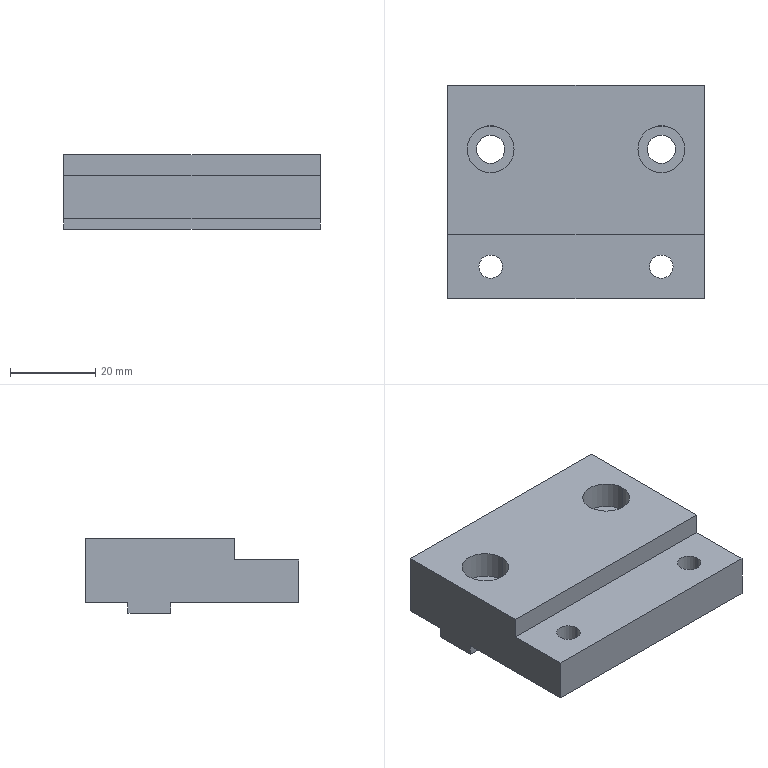Component | SolidWorks | Q1-A12-S21-Q4E.SLDASQ-4_Q1-A12-S21-Q4E-01A-1 | 1 solid | 32 faces | box 60 x 50 x 17.5 mm | volume 38957 mm3 | cylinder 16 | plane 16 | commonest cylinder face diameters 10 x4 5.5 x4 11 x4 6.6 x4 | material Q235-Steel
build123d program:
from build123d import *

# Parameters (mm, degrees)
SKETCH1_W                                       = 60
SKETCH1_H                                       = 50
BOSS_EXTRUDE1_DEPTH                             = 17.5
SKETCH2_W                                       = 5
SKETCH2_H                                       = 15
CUT_EXTRUDE1_DEPTH                              = 68.315
M6_HEX_SOCKET_HEAD_CAP_SCREW_CBORE2_D           = 6.6
M6_HEX_SOCKET_HEAD_CAP_SCREW_CBORE2_CBORE_D     = 11
M6_HEX_SOCKET_HEAD_CAP_SCREW_CBORE2_CBORE_DEPTH = 6.4
SKETCH7_W                                       = 2.5
SKETCH7_H                                       = 10
SKETCH7_H_2                                     = 30
CUT_EXTRUDE2_DEPTH                              = 68.315
M5_HEX_SOCKET_HEAD_CAP_SCREW_CBORE1_D           = 5.5
M5_HEX_SOCKET_HEAD_CAP_SCREW_CBORE1_CBORE_D     = 10
M5_HEX_SOCKET_HEAD_CAP_SCREW_CBORE1_CBORE_DEPTH = 5.4


with BuildPart() as part:
    # Sketch1 → Boss-Extrude1 (new body)
    with BuildSketch(Plane.XY):
        Rectangle(SKETCH1_W, SKETCH1_H)
    extrude(amount=BOSS_EXTRUDE1_DEPTH)

    # Sketch2 → Cut-Extrude1 (cut, through all)
    with BuildSketch(Plane(origin=(30, 0, 0), x_dir=(0, 0, -1), z_dir=(1, 0, 0))):
        with Locations((-15, -17.5)):
            Rectangle(SKETCH2_W, SKETCH2_H)
    extrude(amount=-CUT_EXTRUDE1_DEPTH, mode=Mode.SUBTRACT)

    # M6 Hex Socket Head Cap Screw CBORE2 (through all)
    with Locations(Plane.XY.offset(17.5)):
        with Locations((20, 10), (-20, 10)):
            CounterBoreHole(M6_HEX_SOCKET_HEAD_CAP_SCREW_CBORE2_D / 2, M6_HEX_SOCKET_HEAD_CAP_SCREW_CBORE2_CBORE_D / 2, M6_HEX_SOCKET_HEAD_CAP_SCREW_CBORE2_CBORE_DEPTH)

    # Sketch7 → Cut-Extrude2 (cut, through all)
    with BuildSketch(Plane(origin=(30, 0, 0), x_dir=(0, 0, -1), z_dir=(1, 0, 0))):
        with Locations((-1.25, 20)):
            Rectangle(SKETCH7_W, SKETCH7_H)
        with Locations((-1.25, -10)):
            Rectangle(SKETCH7_W, SKETCH7_H_2)
    extrude(amount=-CUT_EXTRUDE2_DEPTH, mode=Mode.SUBTRACT)

    # M5 Hex Socket Head Cap Screw CBORE1 (through all)
    with Locations(Plane(origin=(0, 0, 2.5), x_dir=(-1, 0, 0), z_dir=(0, 0, -1))):
        with Locations((-20, -17.5), (20, -17.5)):
            CounterBoreHole(M5_HEX_SOCKET_HEAD_CAP_SCREW_CBORE1_D / 2, M5_HEX_SOCKET_HEAD_CAP_SCREW_CBORE1_CBORE_D / 2, M5_HEX_SOCKET_HEAD_CAP_SCREW_CBORE1_CBORE_DEPTH)


solid = part.part

# Placed as in the assembly
solid = solid.moved(Location((1798.5, -30, 147.5), (0, 0, 0)))
STEP:
#1=COLOUR_RGB('',0.7922,0.8196,0.9333);
#2=FILL_AREA_STYLE_COLOUR('',#1);
#3=FILL_AREA_STYLE('',(#2));
#4=SURFACE_STYLE_FILL_AREA(#3);
#5=SURFACE_SIDE_STYLE('',(#4));
#6=SURFACE_STYLE_USAGE(.BOTH.,#5);
#7=PRESENTATION_STYLE_ASSIGNMENT((#6));
#8=CARTESIAN_POINT('',(71.791,-1.87,6.118));
#9=VERTEX_POINT('',#8);
#10=CARTESIAN_POINT('',(71.398,-1.87,6.118));
#11=VERTEX_POINT('',#10);
#12=CARTESIAN_POINT('',(71.594,-1.87,6.118));
#13=DIRECTION('',(0.,0.,-1.));
#14=DIRECTION('',(-1.,0.,0.));
#15=AXIS2_PLACEMENT_3D('',#12,#13,#14);
#16=CIRCLE('',#15,0.1969);
#17=EDGE_CURVE('',#9,#11,#16,.T.);
#18=ORIENTED_EDGE('',*,*,#17,.F.);
#19=CARTESIAN_POINT('',(71.791,-1.87,5.906));
#20=VERTEX_POINT('',#19);
#21=CARTESIAN_POINT('',(71.791,-1.87,5.906));
#22=DIRECTION('',(0.,0.,-1.));
#23=VECTOR('',#22,39.37);
#24=LINE('',#21,#23);
#25=EDGE_CURVE('',#9,#20,#24,.T.);
#26=ORIENTED_EDGE('',*,*,#25,.T.);
#27=CARTESIAN_POINT('',(71.398,-1.87,5.906));
#28=VERTEX_POINT('',#27);
#29=CARTESIAN_POINT('',(71.594,-1.87,5.906));
#30=DIRECTION('',(0.,0.,-1.));
#31=DIRECTION('',(-1.,0.,0.));
#32=AXIS2_PLACEMENT_3D('',#29,#30,#31);
#33=CIRCLE('',#32,0.1969);
#34=EDGE_CURVE('',#20,#28,#33,.T.);
#35=ORIENTED_EDGE('',*,*,#34,.T.);
#36=CARTESIAN_POINT('',(71.398,-1.87,5.906));
#37=DIRECTION('',(0.,0.,-1.));
#38=VECTOR('',#37,39.37);
#39=LINE('',#36,#38);
#40=EDGE_CURVE('',#11,#28,#39,.T.);
#41=ORIENTED_EDGE('',*,*,#40,.F.);
#42=EDGE_LOOP('',(#18,#26,#35,#41));
#43=FACE_OUTER_BOUND('',#42,.T.);
#44=CARTESIAN_POINT('',(71.594,-1.87,5.906));
#45=DIRECTION('',(0.,0.,-1.));
#46=DIRECTION('',(-1.,0.,0.));
#47=AXIS2_PLACEMENT_3D('',#44,#45,#46);
#48=CYLINDRICAL_SURFACE('',#47,0.1969);
#49=ADVANCED_FACE('',(#43),#48,.F.);
#50=CARTESIAN_POINT('',(71.703,-1.87,6.299));
#51=VERTEX_POINT('',#50);
#52=CARTESIAN_POINT('',(71.486,-1.87,6.299));
#53=VERTEX_POINT('',#52);
#54=CARTESIAN_POINT('',(71.594,-1.87,6.299));
#55=DIRECTION('',(0.,0.,-1.));
#56=DIRECTION('',(-1.,0.,0.));
#57=AXIS2_PLACEMENT_3D('',#54,#55,#56);
#58=CIRCLE('',#57,0.1083);
#59=EDGE_CURVE('',#51,#53,#58,.T.);
#60=ORIENTED_EDGE('',*,*,#59,.F.);
#61=CARTESIAN_POINT('',(71.703,-1.87,6.118));
#62=VERTEX_POINT('',#61);
#63=CARTESIAN_POINT('',(71.703,-1.87,5.906));
#64=DIRECTION('',(0.,0.,-1.));
#65=VECTOR('',#64,39.37);
#66=LINE('',#63,#65);
#67=EDGE_CURVE('',#51,#62,#66,.T.);
#68=ORIENTED_EDGE('',*,*,#67,.T.);
#69=CARTESIAN_POINT('',(71.486,-1.87,6.118));
#70=VERTEX_POINT('',#69);
#71=CARTESIAN_POINT('',(71.594,-1.87,6.118));
#72=DIRECTION('',(0.,0.,-1.));
#73=DIRECTION('',(-1.,0.,0.));
#74=AXIS2_PLACEMENT_3D('',#71,#72,#73);
#75=CIRCLE('',#74,0.1083);
#76=EDGE_CURVE('',#62,#70,#75,.T.);
#77=ORIENTED_EDGE('',*,*,#76,.T.);
#78=CARTESIAN_POINT('',(71.486,-1.87,5.906));
#79=DIRECTION('',(0.,0.,-1.));
#80=VECTOR('',#79,39.37);
#81=LINE('',#78,#80);
#82=EDGE_CURVE('',#53,#70,#81,.T.);
#83=ORIENTED_EDGE('',*,*,#82,.F.);
#84=EDGE_LOOP('',(#60,#68,#77,#83));
#85=FACE_OUTER_BOUND('',#84,.T.);
#86=CARTESIAN_POINT('',(71.594,-1.87,5.906));
#87=DIRECTION('',(0.,0.,-1.));
#88=DIRECTION('',(-1.,0.,0.));
#89=AXIS2_PLACEMENT_3D('',#86,#87,#88);
#90=CYLINDRICAL_SURFACE('',#89,0.1083);
#91=ADVANCED_FACE('',(#85),#90,.F.);
#92=CARTESIAN_POINT('',(70.217,-1.87,6.118));
#93=VERTEX_POINT('',#92);
#94=CARTESIAN_POINT('',(69.823,-1.87,6.118));
#95=VERTEX_POINT('',#94);
#96=CARTESIAN_POINT('',(70.02,-1.87,6.118));
#97=DIRECTION('',(0.,0.,-1.));
#98=DIRECTION('',(-1.,0.,0.));
#99=AXIS2_PLACEMENT_3D('',#96,#97,#98);
#100=CIRCLE('',#99,0.1969);
#101=EDGE_CURVE('',#93,#95,#100,.T.);
#102=ORIENTED_EDGE('',*,*,#101,.F.);
#103=CARTESIAN_POINT('',(70.217,-1.87,5.906));
#104=VERTEX_POINT('',#103);
#105=CARTESIAN_POINT('',(70.217,-1.87,5.906));
#106=DIRECTION('',(0.,0.,-1.));
#107=VECTOR('',#106,39.37);
#108=LINE('',#105,#107);
#109=EDGE_CURVE('',#93,#104,#108,.T.);
#110=ORIENTED_EDGE('',*,*,#109,.T.);
#111=CARTESIAN_POINT('',(69.823,-1.87,5.906));
#112=VERTEX_POINT('',#111);
#113=CARTESIAN_POINT('',(70.02,-1.87,5.906));
#114=DIRECTION('',(0.,0.,-1.));
#115=DIRECTION('',(-1.,0.,0.));
#116=AXIS2_PLACEMENT_3D('',#113,#114,#115);
#117=CIRCLE('',#116,0.1969);
#118=EDGE_CURVE('',#104,#112,#117,.T.);
#119=ORIENTED_EDGE('',*,*,#118,.T.);
#120=CARTESIAN_POINT('',(69.823,-1.87,5.906));
#121=DIRECTION('',(0.,0.,-1.));
#122=VECTOR('',#121,39.37);
#123=LINE('',#120,#122);
#124=EDGE_CURVE('',#95,#112,#123,.T.);
#125=ORIENTED_EDGE('',*,*,#124,.F.);
#126=EDGE_LOOP('',(#102,#110,#119,#125));
#127=FACE_OUTER_BOUND('',#126,.T.);
#128=CARTESIAN_POINT('',(70.02,-1.87,5.906));
#129=DIRECTION('',(0.,0.,-1.));
#130=DIRECTION('',(-1.,0.,0.));
#131=AXIS2_PLACEMENT_3D('',#128,#129,#130);
#132=CYLINDRICAL_SURFACE('',#131,0.1969);
#133=ADVANCED_FACE('',(#127),#132,.F.);
#134=CARTESIAN_POINT('',(70.128,-1.87,6.299));
#135=VERTEX_POINT('',#134);
#136=CARTESIAN_POINT('',(69.911,-1.87,6.299));
#137=VERTEX_POINT('',#136);
#138=CARTESIAN_POINT('',(70.02,-1.87,6.299));
#139=DIRECTION('',(0.,0.,-1.));
#140=DIRECTION('',(-1.,0.,0.));
#141=AXIS2_PLACEMENT_3D('',#138,#139,#140);
#142=CIRCLE('',#141,0.1083);
#143=EDGE_CURVE('',#135,#137,#142,.T.);
#144=ORIENTED_EDGE('',*,*,#143,.F.);
#145=CARTESIAN_POINT('',(70.128,-1.87,6.118));
#146=VERTEX_POINT('',#145);
#147=CARTESIAN_POINT('',(70.128,-1.87,5.906));
#148=DIRECTION('',(0.,0.,-1.));
#149=VECTOR('',#148,39.37);
#150=LINE('',#147,#149);
#151=EDGE_CURVE('',#135,#146,#150,.T.);
#152=ORIENTED_EDGE('',*,*,#151,.T.);
#153=CARTESIAN_POINT('',(69.911,-1.87,6.118));
#154=VERTEX_POINT('',#153);
#155=CARTESIAN_POINT('',(70.02,-1.87,6.118));
#156=DIRECTION('',(0.,0.,-1.));
#157=DIRECTION('',(-1.,0.,0.));
#158=AXIS2_PLACEMENT_3D('',#155,#156,#157);
#159=CIRCLE('',#158,0.1083);
#160=EDGE_CURVE('',#146,#154,#159,.T.);
#161=ORIENTED_EDGE('',*,*,#160,.T.);
#162=CARTESIAN_POINT('',(69.911,-1.87,5.906));
#163=DIRECTION('',(0.,0.,-1.));
#164=VECTOR('',#163,39.37);
#165=LINE('',#162,#164);
#166=EDGE_CURVE('',#137,#154,#165,.T.);
#167=ORIENTED_EDGE('',*,*,#166,.F.);
#168=EDGE_LOOP('',(#144,#152,#161,#167));
#169=FACE_OUTER_BOUND('',#168,.T.);
#170=CARTESIAN_POINT('',(70.02,-1.87,5.906));
#171=DIRECTION('',(0.,0.,-1.));
#172=DIRECTION('',(-1.,0.,0.));
#173=AXIS2_PLACEMENT_3D('',#170,#171,#172);
#174=CYLINDRICAL_SURFACE('',#173,0.1083);
#175=ADVANCED_FACE('',(#169),#174,.F.);
#176=CARTESIAN_POINT('',(71.378,-0.7874,6.244));
#177=VERTEX_POINT('',#176);
#178=CARTESIAN_POINT('',(71.811,-0.7874,6.244));
#179=VERTEX_POINT('',#178);
#180=CARTESIAN_POINT('',(71.594,-0.7874,6.244));
#181=DIRECTION('',(0.,0.,1.));
#182=DIRECTION('',(1.,0.,0.));
#183=AXIS2_PLACEMENT_3D('',#180,#181,#182);
#184=CIRCLE('',#183,0.2165);
#185=EDGE_CURVE('',#177,#179,#184,.T.);
#186=ORIENTED_EDGE('',*,*,#185,.F.);
#187=CARTESIAN_POINT('',(71.378,-0.7874,6.496));
#188=VERTEX_POINT('',#187);
#189=CARTESIAN_POINT('',(71.378,-0.7874,6.496));
#190=DIRECTION('',(0.,0.,1.));
#191=VECTOR('',#190,39.37);
#192=LINE('',#189,#191);
#193=EDGE_CURVE('',#177,#188,#192,.T.);
#194=ORIENTED_EDGE('',*,*,#193,.T.);
#195=CARTESIAN_POINT('',(71.811,-0.7874,6.496));
#196=VERTEX_POINT('',#195);
#197=CARTESIAN_POINT('',(71.594,-0.7874,6.496));
#198=DIRECTION('',(0.,0.,1.));
#199=DIRECTION('',(1.,0.,0.));
#200=AXIS2_PLACEMENT_3D('',#197,#198,#199);
#201=CIRCLE('',#200,0.2165);
#202=EDGE_CURVE('',#188,#196,#201,.T.);
#203=ORIENTED_EDGE('',*,*,#202,.T.);
#204=CARTESIAN_POINT('',(71.811,-0.7874,6.496));
#205=DIRECTION('',(0.,0.,1.));
#206=VECTOR('',#205,39.37);
#207=LINE('',#204,#206);
#208=EDGE_CURVE('',#179,#196,#207,.T.);
#209=ORIENTED_EDGE('',*,*,#208,.F.);
#210=EDGE_LOOP('',(#186,#194,#203,#209));
#211=FACE_OUTER_BOUND('',#210,.T.);
#212=CARTESIAN_POINT('',(71.594,-0.7874,6.496));
#213=DIRECTION('',(0.,0.,1.));
#214=DIRECTION('',(1.,0.,0.));
#215=AXIS2_PLACEMENT_3D('',#212,#213,#214);
#216=CYLINDRICAL_SURFACE('',#215,0.2165);
#217=ADVANCED_FACE('',(#211),#216,.F.);
#218=CARTESIAN_POINT('',(71.465,-0.7874,5.807));
#219=VERTEX_POINT('',#218);
#220=CARTESIAN_POINT('',(71.724,-0.7874,5.807));
#221=VERTEX_POINT('',#220);
#222=CARTESIAN_POINT('',(71.594,-0.7874,5.807));
#223=DIRECTION('',(0.,0.,1.));
#224=DIRECTION('',(1.,0.,0.));
#225=AXIS2_PLACEMENT_3D('',#222,#223,#224);
#226=CIRCLE('',#225,0.1299);
#227=EDGE_CURVE('',#219,#221,#226,.T.);
#228=ORIENTED_EDGE('',*,*,#227,.F.);
#229=CARTESIAN_POINT('',(71.465,-0.7874,6.244));
#230=VERTEX_POINT('',#229);
#231=CARTESIAN_POINT('',(71.465,-0.7874,6.496));
#232=DIRECTION('',(0.,0.,1.));
#233=VECTOR('',#232,39.37);
#234=LINE('',#231,#233);
#235=EDGE_CURVE('',#219,#230,#234,.T.);
#236=ORIENTED_EDGE('',*,*,#235,.T.);
#237=CARTESIAN_POINT('',(71.724,-0.7874,6.244));
#238=VERTEX_POINT('',#237);
#239=CARTESIAN_POINT('',(71.594,-0.7874,6.244));
#240=DIRECTION('',(0.,0.,1.));
#241=DIRECTION('',(1.,0.,0.));
#242=AXIS2_PLACEMENT_3D('',#239,#240,#241);
#243=CIRCLE('',#242,0.1299);
#244=EDGE_CURVE('',#230,#238,#243,.T.);
#245=ORIENTED_EDGE('',*,*,#244,.T.);
#246=CARTESIAN_POINT('',(71.724,-0.7874,6.496));
#247=DIRECTION('',(0.,0.,1.));
#248=VECTOR('',#247,39.37);
#249=LINE('',#246,#248);
#250=EDGE_CURVE('',#221,#238,#249,.T.);
#251=ORIENTED_EDGE('',*,*,#250,.F.);
#252=EDGE_LOOP('',(#228,#236,#245,#251));
#253=FACE_OUTER_BOUND('',#252,.T.);
#254=CARTESIAN_POINT('',(71.594,-0.7874,6.496));
#255=DIRECTION('',(0.,0.,1.));
#256=DIRECTION('',(1.,0.,0.));
#257=AXIS2_PLACEMENT_3D('',#254,#255,#256);
#258=CYLINDRICAL_SURFACE('',#257,0.1299);
#259=ADVANCED_FACE('',(#253),#258,.F.);
#260=CARTESIAN_POINT('',(69.803,-0.7874,6.244));
#261=VERTEX_POINT('',#260);
#262=CARTESIAN_POINT('',(70.236,-0.7874,6.244));
#263=VERTEX_POINT('',#262);
#264=CARTESIAN_POINT('',(70.02,-0.7874,6.244));
#265=DIRECTION('',(0.,0.,1.));
#266=DIRECTION('',(1.,0.,0.));
#267=AXIS2_PLACEMENT_3D('',#264,#265,#266);
#268=CIRCLE('',#267,0.2165);
#269=EDGE_CURVE('',#261,#263,#268,.T.);
#270=ORIENTED_EDGE('',*,*,#269,.F.);
#271=CARTESIAN_POINT('',(69.803,-0.7874,6.496));
#272=VERTEX_POINT('',#271);
#273=CARTESIAN_POINT('',(69.803,-0.7874,6.496));
#274=DIRECTION('',(0.,0.,1.));
#275=VECTOR('',#274,39.37);
#276=LINE('',#273,#275);
#277=EDGE_CURVE('',#261,#272,#276,.T.);
#278=ORIENTED_EDGE('',*,*,#277,.T.);
#279=CARTESIAN_POINT('',(70.236,-0.7874,6.496));
#280=VERTEX_POINT('',#279);
#281=CARTESIAN_POINT('',(70.02,-0.7874,6.496));
#282=DIRECTION('',(0.,0.,1.));
#283=DIRECTION('',(1.,0.,0.));
#284=AXIS2_PLACEMENT_3D('',#281,#282,#283);
#285=CIRCLE('',#284,0.2165);
#286=EDGE_CURVE('',#272,#280,#285,.T.);
#287=ORIENTED_EDGE('',*,*,#286,.T.);
#288=CARTESIAN_POINT('',(70.236,-0.7874,6.496));
#289=DIRECTION('',(0.,0.,1.));
#290=VECTOR('',#289,39.37);
#291=LINE('',#288,#290);
#292=EDGE_CURVE('',#263,#280,#291,.T.);
#293=ORIENTED_EDGE('',*,*,#292,.F.);
#294=EDGE_LOOP('',(#270,#278,#287,#293));
#295=FACE_OUTER_BOUND('',#294,.T.);
#296=CARTESIAN_POINT('',(70.02,-0.7874,6.496));
#297=DIRECTION('',(0.,0.,1.));
#298=DIRECTION('',(1.,0.,0.));
#299=AXIS2_PLACEMENT_3D('',#296,#297,#298);
#300=CYLINDRICAL_SURFACE('',#299,0.2165);
#301=ADVANCED_FACE('',(#295),#300,.F.);
#302=CARTESIAN_POINT('',(69.89,-0.7874,5.807));
#303=VERTEX_POINT('',#302);
#304=CARTESIAN_POINT('',(70.15,-0.7874,5.807));
#305=VERTEX_POINT('',#304);
#306=CARTESIAN_POINT('',(70.02,-0.7874,5.807));
#307=DIRECTION('',(0.,0.,1.));
#308=DIRECTION('',(1.,0.,0.));
#309=AXIS2_PLACEMENT_3D('',#306,#307,#308);
#310=CIRCLE('',#309,0.1299);
#311=EDGE_CURVE('',#303,#305,#310,.T.);
#312=ORIENTED_EDGE('',*,*,#311,.F.);
#313=CARTESIAN_POINT('',(69.89,-0.7874,6.244));
#314=VERTEX_POINT('',#313);
#315=CARTESIAN_POINT('',(69.89,-0.7874,6.496));
#316=DIRECTION('',(0.,0.,1.));
#317=VECTOR('',#316,39.37);
#318=LINE('',#315,#317);
#319=EDGE_CURVE('',#303,#314,#318,.T.);
#320=ORIENTED_EDGE('',*,*,#319,.T.);
#321=CARTESIAN_POINT('',(70.15,-0.7874,6.244));
#322=VERTEX_POINT('',#321);
#323=CARTESIAN_POINT('',(70.02,-0.7874,6.244));
#324=DIRECTION('',(0.,0.,1.));
#325=DIRECTION('',(1.,0.,0.));
#326=AXIS2_PLACEMENT_3D('',#323,#324,#325);
#327=CIRCLE('',#326,0.1299);
#328=EDGE_CURVE('',#314,#322,#327,.T.);
#329=ORIENTED_EDGE('',*,*,#328,.T.);
#330=CARTESIAN_POINT('',(70.15,-0.7874,6.496));
#331=DIRECTION('',(0.,0.,1.));
#332=VECTOR('',#331,39.37);
#333=LINE('',#330,#332);
#334=EDGE_CURVE('',#305,#322,#333,.T.);
#335=ORIENTED_EDGE('',*,*,#334,.F.);
#336=EDGE_LOOP('',(#312,#320,#329,#335));
#337=FACE_OUTER_BOUND('',#336,.T.);
#338=CARTESIAN_POINT('',(70.02,-0.7874,6.496));
#339=DIRECTION('',(0.,0.,1.));
#340=DIRECTION('',(1.,0.,0.));
#341=AXIS2_PLACEMENT_3D('',#338,#339,#340);
#342=CYLINDRICAL_SURFACE('',#341,0.1299);
#343=ADVANCED_FACE('',(#337),#342,.F.);
#344=CARTESIAN_POINT('',(71.988,-2.165,6.299));
#345=VERTEX_POINT('',#344);
#346=CARTESIAN_POINT('',(71.988,-2.165,5.906));
#347=VERTEX_POINT('',#346);
#348=CARTESIAN_POINT('',(71.988,-2.165,6.496));
#349=DIRECTION('',(0.,0.,-1.));
#350=VECTOR('',#349,39.37);
#351=LINE('',#348,#350);
#352=EDGE_CURVE('',#345,#347,#351,.T.);
#353=ORIENTED_EDGE('',*,*,#352,.T.);
#354=CARTESIAN_POINT('',(71.988,-0.9843,5.906));
#355=VERTEX_POINT('',#354);
#356=CARTESIAN_POINT('',(71.988,-2.165,5.906));
#357=DIRECTION('',(0.,-1.,0.));
#358=VECTOR('',#357,39.37);
#359=LINE('',#356,#358);
#360=EDGE_CURVE('',#355,#347,#359,.T.);
#361=ORIENTED_EDGE('',*,*,#360,.F.);
#362=CARTESIAN_POINT('',(71.988,-0.9843,5.807));
#363=VERTEX_POINT('',#362);
#364=CARTESIAN_POINT('',(71.988,-0.9843,5.807));
#365=DIRECTION('',(0.,0.,1.));
#366=VECTOR('',#365,39.37);
#367=LINE('',#364,#366);
#368=EDGE_CURVE('',#363,#355,#367,.T.);
#369=ORIENTED_EDGE('',*,*,#368,.F.);
#370=CARTESIAN_POINT('',(71.988,-0.5906,5.807));
#371=VERTEX_POINT('',#370);
#372=CARTESIAN_POINT('',(71.988,-2.165,5.807));
#373=DIRECTION('',(0.,1.,0.));
#374=VECTOR('',#373,39.37);
#375=LINE('',#372,#374);
#376=EDGE_CURVE('',#363,#371,#375,.T.);
#377=ORIENTED_EDGE('',*,*,#376,.T.);
#378=CARTESIAN_POINT('',(71.988,-0.5906,5.906));
#379=VERTEX_POINT('',#378);
#380=CARTESIAN_POINT('',(71.988,-0.5906,5.807));
#381=DIRECTION('',(0.,0.,-1.));
#382=VECTOR('',#381,39.37);
#383=LINE('',#380,#382);
#384=EDGE_CURVE('',#379,#371,#383,.T.);
#385=ORIENTED_EDGE('',*,*,#384,.F.);
#386=CARTESIAN_POINT('',(71.988,-0.1969,5.906));
#387=VERTEX_POINT('',#386);
#388=CARTESIAN_POINT('',(71.988,-0.1969,5.906));
#389=DIRECTION('',(0.,-1.,0.));
#390=VECTOR('',#389,39.37);
#391=LINE('',#388,#390);
#392=EDGE_CURVE('',#387,#379,#391,.T.);
#393=ORIENTED_EDGE('',*,*,#392,.F.);
#394=CARTESIAN_POINT('',(71.988,-0.1969,6.496));
#395=VERTEX_POINT('',#394);
#396=CARTESIAN_POINT('',(71.988,-0.1969,6.496));
#397=DIRECTION('',(0.,0.,-1.));
#398=VECTOR('',#397,39.37);
#399=LINE('',#396,#398);
#400=EDGE_CURVE('',#395,#387,#399,.T.);
#401=ORIENTED_EDGE('',*,*,#400,.F.);
#402=CARTESIAN_POINT('',(71.988,-1.575,6.496));
#403=VERTEX_POINT('',#402);
#404=CARTESIAN_POINT('',(71.988,-2.165,6.496));
#405=DIRECTION('',(0.,1.,0.));
#406=VECTOR('',#405,39.37);
#407=LINE('',#404,#406);
#408=EDGE_CURVE('',#403,#395,#407,.T.);
#409=ORIENTED_EDGE('',*,*,#408,.F.);
#410=CARTESIAN_POINT('',(71.988,-1.575,6.299));
#411=VERTEX_POINT('',#410);
#412=CARTESIAN_POINT('',(71.988,-1.575,6.496));
#413=DIRECTION('',(0.,0.,1.));
#414=VECTOR('',#413,39.37);
#415=LINE('',#412,#414);
#416=EDGE_CURVE('',#411,#403,#415,.T.);
#417=ORIENTED_EDGE('',*,*,#416,.F.);
#418=CARTESIAN_POINT('',(71.988,-2.165,6.299));
#419=DIRECTION('',(0.,1.,0.));
#420=VECTOR('',#419,39.37);
#421=LINE('',#418,#420);
#422=EDGE_CURVE('',#345,#411,#421,.T.);
#423=ORIENTED_EDGE('',*,*,#422,.F.);
#424=EDGE_LOOP('',(#353,#361,#369,#377,#385,#393,#401,#409,#417,#423));
#425=FACE_OUTER_BOUND('',#424,.T.);
#426=CARTESIAN_POINT('',(71.988,-2.165,6.496));
#427=DIRECTION('',(-1.,0.,0.));
#428=DIRECTION('',(0.,0.,1.));
#429=AXIS2_PLACEMENT_3D('',#426,#427,#428);
#430=PLANE('',#429);
#431=ADVANCED_FACE('',(#425),#430,.F.);
#432=ORIENTED_EDGE('',*,*,#400,.T.);
#433=CARTESIAN_POINT('',(69.626,-0.1969,5.906));
#434=VERTEX_POINT('',#433);
#435=CARTESIAN_POINT('',(69.626,-0.1969,5.906));
#436=DIRECTION('',(1.,0.,0.));
#437=VECTOR('',#436,39.37);
#438=LINE('',#435,#437);
#439=EDGE_CURVE('',#434,#387,#438,.T.);
#440=ORIENTED_EDGE('',*,*,#439,.F.);
#441=CARTESIAN_POINT('',(69.626,-0.1969,6.496));
#442=VERTEX_POINT('',#441);
#443=CARTESIAN_POINT('',(69.626,-0.1969,6.496));
#444=DIRECTION('',(0.,0.,-1.));
#445=VECTOR('',#444,39.37);
#446=LINE('',#443,#445);
#447=EDGE_CURVE('',#442,#434,#446,.T.);
#448=ORIENTED_EDGE('',*,*,#447,.F.);
#449=CARTESIAN_POINT('',(69.626,-0.1969,6.496));
#450=DIRECTION('',(-1.,0.,0.));
#451=VECTOR('',#450,39.37);
#452=LINE('',#449,#451);
#453=EDGE_CURVE('',#395,#442,#452,.T.);
#454=ORIENTED_EDGE('',*,*,#453,.F.);
#455=EDGE_LOOP('',(#432,#440,#448,#454));
#456=FACE_OUTER_BOUND('',#455,.T.);
#457=CARTESIAN_POINT('',(69.626,-0.1969,6.496));
#458=DIRECTION('',(0.,-1.,0.));
#459=DIRECTION('',(0.,0.,-1.));
#460=AXIS2_PLACEMENT_3D('',#457,#458,#459);
#461=PLANE('',#460);
#462=ADVANCED_FACE('',(#456),#461,.F.);
#463=CARTESIAN_POINT('',(69.626,-0.9843,5.807));
#464=VERTEX_POINT('',#463);
#465=CARTESIAN_POINT('',(69.626,-0.9843,5.906));
#466=VERTEX_POINT('',#465);
#467=CARTESIAN_POINT('',(69.626,-0.9843,5.807));
#468=DIRECTION('',(0.,0.,1.));
#469=VECTOR('',#468,39.37);
#470=LINE('',#467,#469);
#471=EDGE_CURVE('',#464,#466,#470,.T.);
#472=ORIENTED_EDGE('',*,*,#471,.T.);
#473=CARTESIAN_POINT('',(69.626,-2.165,5.906));
#474=VERTEX_POINT('',#473);
#475=CARTESIAN_POINT('',(69.626,-2.165,5.906));
#476=DIRECTION('',(0.,-1.,0.));
#477=VECTOR('',#476,39.37);
#478=LINE('',#475,#477);
#479=EDGE_CURVE('',#466,#474,#478,.T.);
#480=ORIENTED_EDGE('',*,*,#479,.T.);
#481=CARTESIAN_POINT('',(69.626,-2.165,6.299));
#482=VERTEX_POINT('',#481);
#483=CARTESIAN_POINT('',(69.626,-2.165,6.496));
#484=DIRECTION('',(0.,0.,-1.));
#485=VECTOR('',#484,39.37);
#486=LINE('',#483,#485);
#487=EDGE_CURVE('',#482,#474,#486,.T.);
#488=ORIENTED_EDGE('',*,*,#487,.F.);
#489=CARTESIAN_POINT('',(69.626,-1.575,6.299));
#490=VERTEX_POINT('',#489);
#491=CARTESIAN_POINT('',(69.626,-2.165,6.299));
#492=DIRECTION('',(0.,1.,0.));
#493=VECTOR('',#492,39.37);
#494=LINE('',#491,#493);
#495=EDGE_CURVE('',#482,#490,#494,.T.);
#496=ORIENTED_EDGE('',*,*,#495,.T.);
#497=CARTESIAN_POINT('',(69.626,-1.575,6.496));
#498=VERTEX_POINT('',#497);
#499=CARTESIAN_POINT('',(69.626,-1.575,6.496));
#500=DIRECTION('',(0.,0.,1.));
#501=VECTOR('',#500,39.37);
#502=LINE('',#499,#501);
#503=EDGE_CURVE('',#490,#498,#502,.T.);
#504=ORIENTED_EDGE('',*,*,#503,.T.);
#505=CARTESIAN_POINT('',(69.626,-2.165,6.496));
#506=DIRECTION('',(0.,-1.,0.));
#507=VECTOR('',#506,39.37);
#508=LINE('',#505,#507);
#509=EDGE_CURVE('',#442,#498,#508,.T.);
#510=ORIENTED_EDGE('',*,*,#509,.F.);
#511=ORIENTED_EDGE('',*,*,#447,.T.);
#512=CARTESIAN_POINT('',(69.626,-0.5906,5.906));
#513=VERTEX_POINT('',#512);
#514=CARTESIAN_POINT('',(69.626,-0.1969,5.906));
#515=DIRECTION('',(0.,-1.,0.));
#516=VECTOR('',#515,39.37);
#517=LINE('',#514,#516);
#518=EDGE_CURVE('',#434,#513,#517,.T.);
#519=ORIENTED_EDGE('',*,*,#518,.T.);
#520=CARTESIAN_POINT('',(69.626,-0.5906,5.807));
#521=VERTEX_POINT('',#520);
#522=CARTESIAN_POINT('',(69.626,-0.5906,5.807));
#523=DIRECTION('',(0.,0.,-1.));
#524=VECTOR('',#523,39.37);
#525=LINE('',#522,#524);
#526=EDGE_CURVE('',#513,#521,#525,.T.);
#527=ORIENTED_EDGE('',*,*,#526,.T.);
#528=CARTESIAN_POINT('',(69.626,-2.165,5.807));
#529=DIRECTION('',(0.,-1.,0.));
#530=VECTOR('',#529,39.37);
#531=LINE('',#528,#530);
#532=EDGE_CURVE('',#521,#464,#531,.T.);
#533=ORIENTED_EDGE('',*,*,#532,.T.);
#534=EDGE_LOOP('',(#472,#480,#488,#496,#504,#510,#511,#519,#527,#533));
#535=FACE_OUTER_BOUND('',#534,.T.);
#536=CARTESIAN_POINT('',(69.626,-2.165,6.496));
#537=DIRECTION('',(1.,0.,0.));
#538=DIRECTION('',(0.,0.,-1.));
#539=AXIS2_PLACEMENT_3D('',#536,#537,#538);
#540=PLANE('',#539);
#541=ADVANCED_FACE('',(#535),#540,.F.);
#542=ORIENTED_EDGE('',*,*,#487,.T.);
#543=CARTESIAN_POINT('',(69.626,-2.165,5.906));
#544=DIRECTION('',(1.,0.,0.));
#545=VECTOR('',#544,39.37);
#546=LINE('',#543,#545);
#547=EDGE_CURVE('',#474,#347,#546,.T.);
#548=ORIENTED_EDGE('',*,*,#547,.T.);
#549=ORIENTED_EDGE('',*,*,#352,.F.);
#550=CARTESIAN_POINT('',(69.626,-2.165,6.299));
#551=DIRECTION('',(1.,0.,0.));
#552=VECTOR('',#551,39.37);
#553=LINE('',#550,#552);
#554=EDGE_CURVE('',#482,#345,#553,.T.);
#555=ORIENTED_EDGE('',*,*,#554,.F.);
#556=EDGE_LOOP('',(#542,#548,#549,#555));
#557=FACE_OUTER_BOUND('',#556,.T.);
#558=CARTESIAN_POINT('',(69.626,-2.165,6.496));
#559=DIRECTION('',(0.,1.,0.));
#560=DIRECTION('',(0.,0.,1.));
#561=AXIS2_PLACEMENT_3D('',#558,#559,#560);
#562=PLANE('',#561);
#563=ADVANCED_FACE('',(#557),#562,.F.);
#564=CARTESIAN_POINT('',(71.594,-0.7874,6.496));
#565=DIRECTION('',(0.,0.,1.));
#566=DIRECTION('',(1.,0.,0.));
#567=AXIS2_PLACEMENT_3D('',#564,#565,#566);
#568=CIRCLE('',#567,0.2165);
#569=EDGE_CURVE('',#196,#188,#568,.T.);
#570=ORIENTED_EDGE('',*,*,#569,.F.);
#571=ORIENTED_EDGE('',*,*,#202,.F.);
#572=EDGE_LOOP('',(#570,#571));
#573=FACE_BOUND('',#572,.T.);
#574=CARTESIAN_POINT('',(70.02,-0.7874,6.496));
#575=DIRECTION('',(0.,0.,1.));
#576=DIRECTION('',(1.,0.,0.));
#577=AXIS2_PLACEMENT_3D('',#574,#575,#576);
#578=CIRCLE('',#577,0.2165);
#579=EDGE_CURVE('',#280,#272,#578,.T.);
#580=ORIENTED_EDGE('',*,*,#579,.F.);
#581=ORIENTED_EDGE('',*,*,#286,.F.);
#582=EDGE_LOOP('',(#580,#581));
#583=FACE_BOUND('',#582,.T.);
#584=ORIENTED_EDGE('',*,*,#509,.T.);
#585=CARTESIAN_POINT('',(69.626,-1.575,6.496));
#586=DIRECTION('',(1.,0.,0.));
#587=VECTOR('',#586,39.37);
#588=LINE('',#585,#587);
#589=EDGE_CURVE('',#498,#403,#588,.T.);
#590=ORIENTED_EDGE('',*,*,#589,.T.);
#591=ORIENTED_EDGE('',*,*,#408,.T.);
#592=ORIENTED_EDGE('',*,*,#453,.T.);
#593=EDGE_LOOP('',(#584,#590,#591,#592));
#594=FACE_OUTER_BOUND('',#593,.T.);
#595=CARTESIAN_POINT('',(70.807,-1.181,6.496));
#596=DIRECTION('',(0.,0.,-1.));
#597=DIRECTION('',(-1.,0.,0.));
#598=AXIS2_PLACEMENT_3D('',#595,#596,#597);
#599=PLANE('',#598);
#600=ADVANCED_FACE('',(#573,#583,#594),#599,.F.);
#601=CARTESIAN_POINT('',(69.626,-0.9843,5.807));
#602=DIRECTION('',(1.,0.,0.));
#603=VECTOR('',#602,39.37);
#604=LINE('',#601,#603);
#605=EDGE_CURVE('',#464,#363,#604,.T.);
#606=ORIENTED_EDGE('',*,*,#605,.F.);
#607=ORIENTED_EDGE('',*,*,#532,.F.);
#608=CARTESIAN_POINT('',(69.626,-0.5906,5.807));
#609=DIRECTION('',(1.,0.,0.));
#610=VECTOR('',#609,39.37);
#611=LINE('',#608,#610);
#612=EDGE_CURVE('',#521,#371,#611,.T.);
#613=ORIENTED_EDGE('',*,*,#612,.T.);
#614=ORIENTED_EDGE('',*,*,#376,.F.);
#615=EDGE_LOOP('',(#606,#607,#613,#614));
#616=FACE_OUTER_BOUND('',#615,.T.);
#617=CARTESIAN_POINT('',(71.594,-0.7874,5.807));
#618=DIRECTION('',(0.,0.,1.));
#619=DIRECTION('',(1.,0.,0.));
#620=AXIS2_PLACEMENT_3D('',#617,#618,#619);
#621=CIRCLE('',#620,0.1299);
#622=EDGE_CURVE('',#221,#219,#621,.T.);
#623=ORIENTED_EDGE('',*,*,#622,.T.);
#624=ORIENTED_EDGE('',*,*,#227,.T.);
#625=EDGE_LOOP('',(#623,#624));
#626=FACE_BOUND('',#625,.T.);
#627=CARTESIAN_POINT('',(70.02,-0.7874,5.807));
#628=DIRECTION('',(0.,0.,1.));
#629=DIRECTION('',(1.,0.,0.));
#630=AXIS2_PLACEMENT_3D('',#627,#628,#629);
#631=CIRCLE('',#630,0.1299);
#632=EDGE_CURVE('',#305,#303,#631,.T.);
#633=ORIENTED_EDGE('',*,*,#632,.T.);
#634=ORIENTED_EDGE('',*,*,#311,.T.);
#635=EDGE_LOOP('',(#633,#634));
#636=FACE_BOUND('',#635,.T.);
#637=CARTESIAN_POINT('',(70.807,-1.181,5.807));
#638=DIRECTION('',(0.,0.,-1.));
#639=DIRECTION('',(-1.,0.,0.));
#640=AXIS2_PLACEMENT_3D('',#637,#638,#639);
#641=PLANE('',#640);
#642=ADVANCED_FACE('',(#616,#626,#636),#641,.T.);
#643=ORIENTED_EDGE('',*,*,#416,.T.);
#644=ORIENTED_EDGE('',*,*,#589,.F.);
#645=ORIENTED_EDGE('',*,*,#503,.F.);
#646=CARTESIAN_POINT('',(69.626,-1.575,6.299));
#647=DIRECTION('',(1.,0.,0.));
#648=VECTOR('',#647,39.37);
#649=LINE('',#646,#648);
#650=EDGE_CURVE('',#490,#411,#649,.T.);
#651=ORIENTED_EDGE('',*,*,#650,.T.);
#652=EDGE_LOOP('',(#643,#644,#645,#651));
#653=FACE_OUTER_BOUND('',#652,.T.);
#654=CARTESIAN_POINT('',(69.626,-1.575,6.496));
#655=DIRECTION('',(0.,1.,0.));
#656=DIRECTION('',(0.,0.,1.));
#657=AXIS2_PLACEMENT_3D('',#654,#655,#656);
#658=PLANE('',#657);
#659=ADVANCED_FACE('',(#653),#658,.F.);
#660=CARTESIAN_POINT('',(71.594,-1.87,6.299));
#661=DIRECTION('',(0.,0.,-1.));
#662=DIRECTION('',(-1.,0.,0.));
#663=AXIS2_PLACEMENT_3D('',#660,#661,#662);
#664=CIRCLE('',#663,0.1083);
#665=EDGE_CURVE('',#53,#51,#664,.T.);
#666=ORIENTED_EDGE('',*,*,#665,.T.);
#667=ORIENTED_EDGE('',*,*,#59,.T.);
#668=EDGE_LOOP('',(#666,#667));
#669=FACE_BOUND('',#668,.T.);
#670=CARTESIAN_POINT('',(70.02,-1.87,6.299));
#671=DIRECTION('',(0.,0.,-1.));
#672=DIRECTION('',(-1.,0.,0.));
#673=AXIS2_PLACEMENT_3D('',#670,#671,#672);
#674=CIRCLE('',#673,0.1083);
#675=EDGE_CURVE('',#137,#135,#674,.T.);
#676=ORIENTED_EDGE('',*,*,#675,.T.);
#677=ORIENTED_EDGE('',*,*,#143,.T.);
#678=EDGE_LOOP('',(#676,#677));
#679=FACE_BOUND('',#678,.T.);
#680=ORIENTED_EDGE('',*,*,#422,.T.);
#681=ORIENTED_EDGE('',*,*,#650,.F.);
#682=ORIENTED_EDGE('',*,*,#495,.F.);
#683=ORIENTED_EDGE('',*,*,#554,.T.);
#684=EDGE_LOOP('',(#680,#681,#682,#683));
#685=FACE_OUTER_BOUND('',#684,.T.);
#686=CARTESIAN_POINT('',(69.626,-2.165,6.299));
#687=DIRECTION('',(0.,0.,-1.));
#688=DIRECTION('',(-1.,0.,0.));
#689=AXIS2_PLACEMENT_3D('',#686,#687,#688);
#690=PLANE('',#689);
#691=ADVANCED_FACE('',(#669,#679,#685),#690,.F.);
#692=ORIENTED_EDGE('',*,*,#319,.F.);
#693=ORIENTED_EDGE('',*,*,#632,.F.);
#694=ORIENTED_EDGE('',*,*,#334,.T.);
#695=CARTESIAN_POINT('',(70.02,-0.7874,6.244));
#696=DIRECTION('',(0.,0.,1.));
#697=DIRECTION('',(1.,0.,0.));
#698=AXIS2_PLACEMENT_3D('',#695,#696,#697);
#699=CIRCLE('',#698,0.1299);
#700=EDGE_CURVE('',#322,#314,#699,.T.);
#701=ORIENTED_EDGE('',*,*,#700,.T.);
#702=EDGE_LOOP('',(#692,#693,#694,#701));
#703=FACE_OUTER_BOUND('',#702,.T.);
#704=CARTESIAN_POINT('',(70.02,-0.7874,6.496));
#705=DIRECTION('',(0.,0.,1.));
#706=DIRECTION('',(1.,0.,0.));
#707=AXIS2_PLACEMENT_3D('',#704,#705,#706);
#708=CYLINDRICAL_SURFACE('',#707,0.1299);
#709=ADVANCED_FACE('',(#703),#708,.F.);
#710=ORIENTED_EDGE('',*,*,#700,.F.);
#711=ORIENTED_EDGE('',*,*,#328,.F.);
#712=EDGE_LOOP('',(#710,#711));
#713=FACE_BOUND('',#712,.T.);
#714=CARTESIAN_POINT('',(70.02,-0.7874,6.244));
#715=DIRECTION('',(0.,0.,1.));
#716=DIRECTION('',(1.,0.,0.));
#717=AXIS2_PLACEMENT_3D('',#714,#715,#716);
#718=CIRCLE('',#717,0.2165);
#719=EDGE_CURVE('',#263,#261,#718,.T.);
#720=ORIENTED_EDGE('',*,*,#719,.T.);
#721=ORIENTED_EDGE('',*,*,#269,.T.);
#722=EDGE_LOOP('',(#720,#721));
#723=FACE_OUTER_BOUND('',#722,.T.);
#724=CARTESIAN_POINT('',(70.15,-0.7874,6.244));
#725=DIRECTION('',(0.,0.,-1.));
#726=DIRECTION('',(-1.,0.,0.));
#727=AXIS2_PLACEMENT_3D('',#724,#725,#726);
#728=PLANE('',#727);
#729=ADVANCED_FACE('',(#713,#723),#728,.F.);
#730=ORIENTED_EDGE('',*,*,#277,.F.);
#731=ORIENTED_EDGE('',*,*,#719,.F.);
#732=ORIENTED_EDGE('',*,*,#292,.T.);
#733=ORIENTED_EDGE('',*,*,#579,.T.);
#734=EDGE_LOOP('',(#730,#731,#732,#733));
#735=FACE_OUTER_BOUND('',#734,.T.);
#736=CARTESIAN_POINT('',(70.02,-0.7874,6.496));
#737=DIRECTION('',(0.,0.,1.));
#738=DIRECTION('',(1.,0.,0.));
#739=AXIS2_PLACEMENT_3D('',#736,#737,#738);
#740=CYLINDRICAL_SURFACE('',#739,0.2165);
#741=ADVANCED_FACE('',(#735),#740,.F.);
#742=ORIENTED_EDGE('',*,*,#235,.F.);
#743=ORIENTED_EDGE('',*,*,#622,.F.);
#744=ORIENTED_EDGE('',*,*,#250,.T.);
#745=CARTESIAN_POINT('',(71.594,-0.7874,6.244));
#746=DIRECTION('',(0.,0.,1.));
#747=DIRECTION('',(1.,0.,0.));
#748=AXIS2_PLACEMENT_3D('',#745,#746,#747);
#749=CIRCLE('',#748,0.1299);
#750=EDGE_CURVE('',#238,#230,#749,.T.);
#751=ORIENTED_EDGE('',*,*,#750,.T.);
#752=EDGE_LOOP('',(#742,#743,#744,#751));
#753=FACE_OUTER_BOUND('',#752,.T.);
#754=CARTESIAN_POINT('',(71.594,-0.7874,6.496));
#755=DIRECTION('',(0.,0.,1.));
#756=DIRECTION('',(1.,0.,0.));
#757=AXIS2_PLACEMENT_3D('',#754,#755,#756);
#758=CYLINDRICAL_SURFACE('',#757,0.1299);
#759=ADVANCED_FACE('',(#753),#758,.F.);
#760=ORIENTED_EDGE('',*,*,#750,.F.);
#761=ORIENTED_EDGE('',*,*,#244,.F.);
#762=EDGE_LOOP('',(#760,#761));
#763=FACE_BOUND('',#762,.T.);
#764=CARTESIAN_POINT('',(71.594,-0.7874,6.244));
#765=DIRECTION('',(0.,0.,1.));
#766=DIRECTION('',(1.,0.,0.));
#767=AXIS2_PLACEMENT_3D('',#764,#765,#766);
#768=CIRCLE('',#767,0.2165);
#769=EDGE_CURVE('',#179,#177,#768,.T.);
#770=ORIENTED_EDGE('',*,*,#769,.T.);
#771=ORIENTED_EDGE('',*,*,#185,.T.);
#772=EDGE_LOOP('',(#770,#771));
#773=FACE_OUTER_BOUND('',#772,.T.);
#774=CARTESIAN_POINT('',(71.724,-0.7874,6.244));
#775=DIRECTION('',(0.,0.,-1.));
#776=DIRECTION('',(-1.,0.,0.));
#777=AXIS2_PLACEMENT_3D('',#774,#775,#776);
#778=PLANE('',#777);
#779=ADVANCED_FACE('',(#763,#773),#778,.F.);
#780=ORIENTED_EDGE('',*,*,#193,.F.);
#781=ORIENTED_EDGE('',*,*,#769,.F.);
#782=ORIENTED_EDGE('',*,*,#208,.T.);
#783=ORIENTED_EDGE('',*,*,#569,.T.);
#784=EDGE_LOOP('',(#780,#781,#782,#783));
#785=FACE_OUTER_BOUND('',#784,.T.);
#786=CARTESIAN_POINT('',(71.594,-0.7874,6.496));
#787=DIRECTION('',(0.,0.,1.));
#788=DIRECTION('',(1.,0.,0.));
#789=AXIS2_PLACEMENT_3D('',#786,#787,#788);
#790=CYLINDRICAL_SURFACE('',#789,0.2165);
#791=ADVANCED_FACE('',(#785),#790,.F.);
#792=ORIENTED_EDGE('',*,*,#384,.T.);
#793=ORIENTED_EDGE('',*,*,#612,.F.);
#794=ORIENTED_EDGE('',*,*,#526,.F.);
#795=CARTESIAN_POINT('',(69.626,-0.5906,5.906));
#796=DIRECTION('',(1.,0.,0.));
#797=VECTOR('',#796,39.37);
#798=LINE('',#795,#797);
#799=EDGE_CURVE('',#513,#379,#798,.T.);
#800=ORIENTED_EDGE('',*,*,#799,.T.);
#801=EDGE_LOOP('',(#792,#793,#794,#800));
#802=FACE_OUTER_BOUND('',#801,.T.);
#803=CARTESIAN_POINT('',(69.626,-0.5906,5.807));
#804=DIRECTION('',(0.,-1.,-0.));
#805=DIRECTION('',(0.,0.,-1.));
#806=AXIS2_PLACEMENT_3D('',#803,#804,#805);
#807=PLANE('',#806);
#808=ADVANCED_FACE('',(#802),#807,.F.);
#809=ORIENTED_EDGE('',*,*,#392,.T.);
#810=ORIENTED_EDGE('',*,*,#799,.F.);
#811=ORIENTED_EDGE('',*,*,#518,.F.);
#812=ORIENTED_EDGE('',*,*,#439,.T.);
#813=EDGE_LOOP('',(#809,#810,#811,#812));
#814=FACE_OUTER_BOUND('',#813,.T.);
#815=CARTESIAN_POINT('',(69.626,-0.1969,5.906));
#816=DIRECTION('',(0.,0.,1.));
#817=DIRECTION('',(0.,-1.,0.));
#818=AXIS2_PLACEMENT_3D('',#815,#816,#817);
#819=PLANE('',#818);
#820=ADVANCED_FACE('',(#814),#819,.F.);
#821=CARTESIAN_POINT('',(71.594,-1.87,5.906));
#822=DIRECTION('',(0.,0.,-1.));
#823=DIRECTION('',(-1.,0.,0.));
#824=AXIS2_PLACEMENT_3D('',#821,#822,#823);
#825=CIRCLE('',#824,0.1969);
#826=EDGE_CURVE('',#28,#20,#825,.T.);
#827=ORIENTED_EDGE('',*,*,#826,.F.);
#828=ORIENTED_EDGE('',*,*,#34,.F.);
#829=EDGE_LOOP('',(#827,#828));
#830=FACE_BOUND('',#829,.T.);
#831=CARTESIAN_POINT('',(70.02,-1.87,5.906));
#832=DIRECTION('',(0.,0.,-1.));
#833=DIRECTION('',(-1.,0.,0.));
#834=AXIS2_PLACEMENT_3D('',#831,#832,#833);
#835=CIRCLE('',#834,0.1969);
#836=EDGE_CURVE('',#112,#104,#835,.T.);
#837=ORIENTED_EDGE('',*,*,#836,.F.);
#838=ORIENTED_EDGE('',*,*,#118,.F.);
#839=EDGE_LOOP('',(#837,#838));
#840=FACE_BOUND('',#839,.T.);
#841=ORIENTED_EDGE('',*,*,#360,.T.);
#842=ORIENTED_EDGE('',*,*,#547,.F.);
#843=ORIENTED_EDGE('',*,*,#479,.F.);
#844=CARTESIAN_POINT('',(69.626,-0.9843,5.906));
#845=DIRECTION('',(1.,0.,0.));
#846=VECTOR('',#845,39.37);
#847=LINE('',#844,#846);
#848=EDGE_CURVE('',#466,#355,#847,.T.);
#849=ORIENTED_EDGE('',*,*,#848,.T.);
#850=EDGE_LOOP('',(#841,#842,#843,#849));
#851=FACE_OUTER_BOUND('',#850,.T.);
#852=CARTESIAN_POINT('',(69.626,-2.165,5.906));
#853=DIRECTION('',(0.,0.,1.));
#854=DIRECTION('',(1.,0.,0.));
#855=AXIS2_PLACEMENT_3D('',#852,#853,#854);
#856=PLANE('',#855);
#857=ADVANCED_FACE('',(#830,#840,#851),#856,.F.);
#858=ORIENTED_EDGE('',*,*,#368,.T.);
#859=ORIENTED_EDGE('',*,*,#848,.F.);
#860=ORIENTED_EDGE('',*,*,#471,.F.);
#861=ORIENTED_EDGE('',*,*,#605,.T.);
#862=EDGE_LOOP('',(#858,#859,#860,#861));
#863=FACE_OUTER_BOUND('',#862,.T.);
#864=CARTESIAN_POINT('',(69.626,-0.9843,5.807));
#865=DIRECTION('',(0.,1.,0.));
#866=DIRECTION('',(0.,0.,1.));
#867=AXIS2_PLACEMENT_3D('',#864,#865,#866);
#868=PLANE('',#867);
#869=ADVANCED_FACE('',(#863),#868,.F.);
#870=ORIENTED_EDGE('',*,*,#151,.F.);
#871=ORIENTED_EDGE('',*,*,#675,.F.);
#872=ORIENTED_EDGE('',*,*,#166,.T.);
#873=CARTESIAN_POINT('',(70.02,-1.87,6.118));
#874=DIRECTION('',(0.,0.,-1.));
#875=DIRECTION('',(-1.,0.,0.));
#876=AXIS2_PLACEMENT_3D('',#873,#874,#875);
#877=CIRCLE('',#876,0.1083);
#878=EDGE_CURVE('',#154,#146,#877,.T.);
#879=ORIENTED_EDGE('',*,*,#878,.T.);
#880=EDGE_LOOP('',(#870,#871,#872,#879));
#881=FACE_OUTER_BOUND('',#880,.T.);
#882=CARTESIAN_POINT('',(70.02,-1.87,5.906));
#883=DIRECTION('',(0.,0.,-1.));
#884=DIRECTION('',(-1.,0.,0.));
#885=AXIS2_PLACEMENT_3D('',#882,#883,#884);
#886=CYLINDRICAL_SURFACE('',#885,0.1083);
#887=ADVANCED_FACE('',(#881),#886,.F.);
#888=ORIENTED_EDGE('',*,*,#878,.F.);
#889=ORIENTED_EDGE('',*,*,#160,.F.);
#890=EDGE_LOOP('',(#888,#889));
#891=FACE_BOUND('',#890,.T.);
#892=CARTESIAN_POINT('',(70.02,-1.87,6.118));
#893=DIRECTION('',(0.,0.,-1.));
#894=DIRECTION('',(-1.,0.,0.));
#895=AXIS2_PLACEMENT_3D('',#892,#893,#894);
#896=CIRCLE('',#895,0.1969);
#897=EDGE_CURVE('',#95,#93,#896,.T.);
#898=ORIENTED_EDGE('',*,*,#897,.T.);
#899=ORIENTED_EDGE('',*,*,#101,.T.);
#900=EDGE_LOOP('',(#898,#899));
#901=FACE_OUTER_BOUND('',#900,.T.);
#902=CARTESIAN_POINT('',(70.128,-1.87,6.118));
#903=DIRECTION('',(0.,0.,1.));
#904=DIRECTION('',(1.,0.,0.));
#905=AXIS2_PLACEMENT_3D('',#902,#903,#904);
#906=PLANE('',#905);
#907=ADVANCED_FACE('',(#891,#901),#906,.F.);
#908=ORIENTED_EDGE('',*,*,#109,.F.);
#909=ORIENTED_EDGE('',*,*,#897,.F.);
#910=ORIENTED_EDGE('',*,*,#124,.T.);
#911=ORIENTED_EDGE('',*,*,#836,.T.);
#912=EDGE_LOOP('',(#908,#909,#910,#911));
#913=FACE_OUTER_BOUND('',#912,.T.);
#914=CARTESIAN_POINT('',(70.02,-1.87,5.906));
#915=DIRECTION('',(0.,0.,-1.));
#916=DIRECTION('',(-1.,0.,0.));
#917=AXIS2_PLACEMENT_3D('',#914,#915,#916);
#918=CYLINDRICAL_SURFACE('',#917,0.1969);
#919=ADVANCED_FACE('',(#913),#918,.F.);
#920=ORIENTED_EDGE('',*,*,#67,.F.);
#921=ORIENTED_EDGE('',*,*,#665,.F.);
#922=ORIENTED_EDGE('',*,*,#82,.T.);
#923=CARTESIAN_POINT('',(71.594,-1.87,6.118));
#924=DIRECTION('',(0.,0.,-1.));
#925=DIRECTION('',(-1.,0.,0.));
#926=AXIS2_PLACEMENT_3D('',#923,#924,#925);
#927=CIRCLE('',#926,0.1083);
#928=EDGE_CURVE('',#70,#62,#927,.T.);
#929=ORIENTED_EDGE('',*,*,#928,.T.);
#930=EDGE_LOOP('',(#920,#921,#922,#929));
#931=FACE_OUTER_BOUND('',#930,.T.);
#932=CARTESIAN_POINT('',(71.594,-1.87,5.906));
#933=DIRECTION('',(0.,0.,-1.));
#934=DIRECTION('',(-1.,0.,0.));
#935=AXIS2_PLACEMENT_3D('',#932,#933,#934);
#936=CYLINDRICAL_SURFACE('',#935,0.1083);
#937=ADVANCED_FACE('',(#931),#936,.F.);
#938=ORIENTED_EDGE('',*,*,#928,.F.);
#939=ORIENTED_EDGE('',*,*,#76,.F.);
#940=EDGE_LOOP('',(#938,#939));
#941=FACE_BOUND('',#940,.T.);
#942=CARTESIAN_POINT('',(71.594,-1.87,6.118));
#943=DIRECTION('',(0.,0.,-1.));
#944=DIRECTION('',(-1.,0.,0.));
#945=AXIS2_PLACEMENT_3D('',#942,#943,#944);
#946=CIRCLE('',#945,0.1969);
#947=EDGE_CURVE('',#11,#9,#946,.T.);
#948=ORIENTED_EDGE('',*,*,#947,.T.);
#949=ORIENTED_EDGE('',*,*,#17,.T.);
#950=EDGE_LOOP('',(#948,#949));
#951=FACE_OUTER_BOUND('',#950,.T.);
#952=CARTESIAN_POINT('',(71.703,-1.87,6.118));
#953=DIRECTION('',(0.,0.,1.));
#954=DIRECTION('',(1.,0.,0.));
#955=AXIS2_PLACEMENT_3D('',#952,#953,#954);
#956=PLANE('',#955);
#957=ADVANCED_FACE('',(#941,#951),#956,.F.);
#958=ORIENTED_EDGE('',*,*,#25,.F.);
#959=ORIENTED_EDGE('',*,*,#947,.F.);
#960=ORIENTED_EDGE('',*,*,#40,.T.);
#961=ORIENTED_EDGE('',*,*,#826,.T.);
#962=EDGE_LOOP('',(#958,#959,#960,#961));
#963=FACE_OUTER_BOUND('',#962,.T.);
#964=CARTESIAN_POINT('',(71.594,-1.87,5.906));
#965=DIRECTION('',(0.,0.,-1.));
#966=DIRECTION('',(-1.,0.,0.));
#967=AXIS2_PLACEMENT_3D('',#964,#965,#966);
#968=CYLINDRICAL_SURFACE('',#967,0.1969);
#969=ADVANCED_FACE('',(#963),#968,.F.);
#970=CLOSED_SHELL('',(#49,#91,#133,#175,#217,#259,#301,#343,#431,#462,#541,#563,#600,#642,#659,#691,#709,#729,#741,#759,#779,#791,#808,#820,#857,#869,#887,#907,#919,#937,#957,#969));
#971=MANIFOLD_SOLID_BREP('',#970);
#972=STYLED_ITEM('',(#7),#971);
#973=(LENGTH_UNIT()NAMED_UNIT(*)SI_UNIT($,.METRE.));
#974=LENGTH_MEASURE_WITH_UNIT(LENGTH_MEASURE(0.0254),#973);
#975=DIMENSIONAL_EXPONENTS(1.,0.,0.,0.,0.,0.,0.);
#976=(CONVERSION_BASED_UNIT('',#974)LENGTH_UNIT()NAMED_UNIT(#975));
#977=UNCERTAINTY_MEASURE_WITH_UNIT(LENGTH_MEASURE(0.00001),#976,'','');
#978=(NAMED_UNIT(*)PLANE_ANGLE_UNIT()SI_UNIT($,.RADIAN.));
#979=(NAMED_UNIT(*)SI_UNIT($,.STERADIAN.)SOLID_ANGLE_UNIT());
#980=(GEOMETRIC_REPRESENTATION_CONTEXT(3)GLOBAL_UNCERTAINTY_ASSIGNED_CONTEXT((#977))GLOBAL_UNIT_ASSIGNED_CONTEXT((#976,#978,#979))REPRESENTATION_CONTEXT('',''));
#981=MECHANICAL_DESIGN_GEOMETRIC_PRESENTATION_REPRESENTATION('',(#972),#980);
#982=PRESENTATION_LAYER_ASSIGNMENT('','',(#972));
#983=CARTESIAN_POINT('',(0.,0.,0.));
#984=DIRECTION('',(0.,0.,1.));
#985=DIRECTION('',(1.,0.,0.));
#986=AXIS2_PLACEMENT_3D('',#983,#984,#985);
#987=(LENGTH_UNIT()NAMED_UNIT(*)SI_UNIT($,.METRE.));
#988=LENGTH_MEASURE_WITH_UNIT(LENGTH_MEASURE(0.0254),#987);
#989=DIMENSIONAL_EXPONENTS(1.,0.,0.,0.,0.,0.,0.);
#990=(CONVERSION_BASED_UNIT('',#988)LENGTH_UNIT()NAMED_UNIT(#989));
#991=UNCERTAINTY_MEASURE_WITH_UNIT(LENGTH_MEASURE(0.00001),#990,'','');
#992=(NAMED_UNIT(*)PLANE_ANGLE_UNIT()SI_UNIT($,.RADIAN.));
#993=(NAMED_UNIT(*)SI_UNIT($,.STERADIAN.)SOLID_ANGLE_UNIT());
#994=(GEOMETRIC_REPRESENTATION_CONTEXT(3)GLOBAL_UNCERTAINTY_ASSIGNED_CONTEXT((#991))GLOBAL_UNIT_ASSIGNED_CONTEXT((#990,#992,#993))REPRESENTATION_CONTEXT('',''));
#995=ADVANCED_BREP_SHAPE_REPRESENTATION('',(#971,#986),#994);